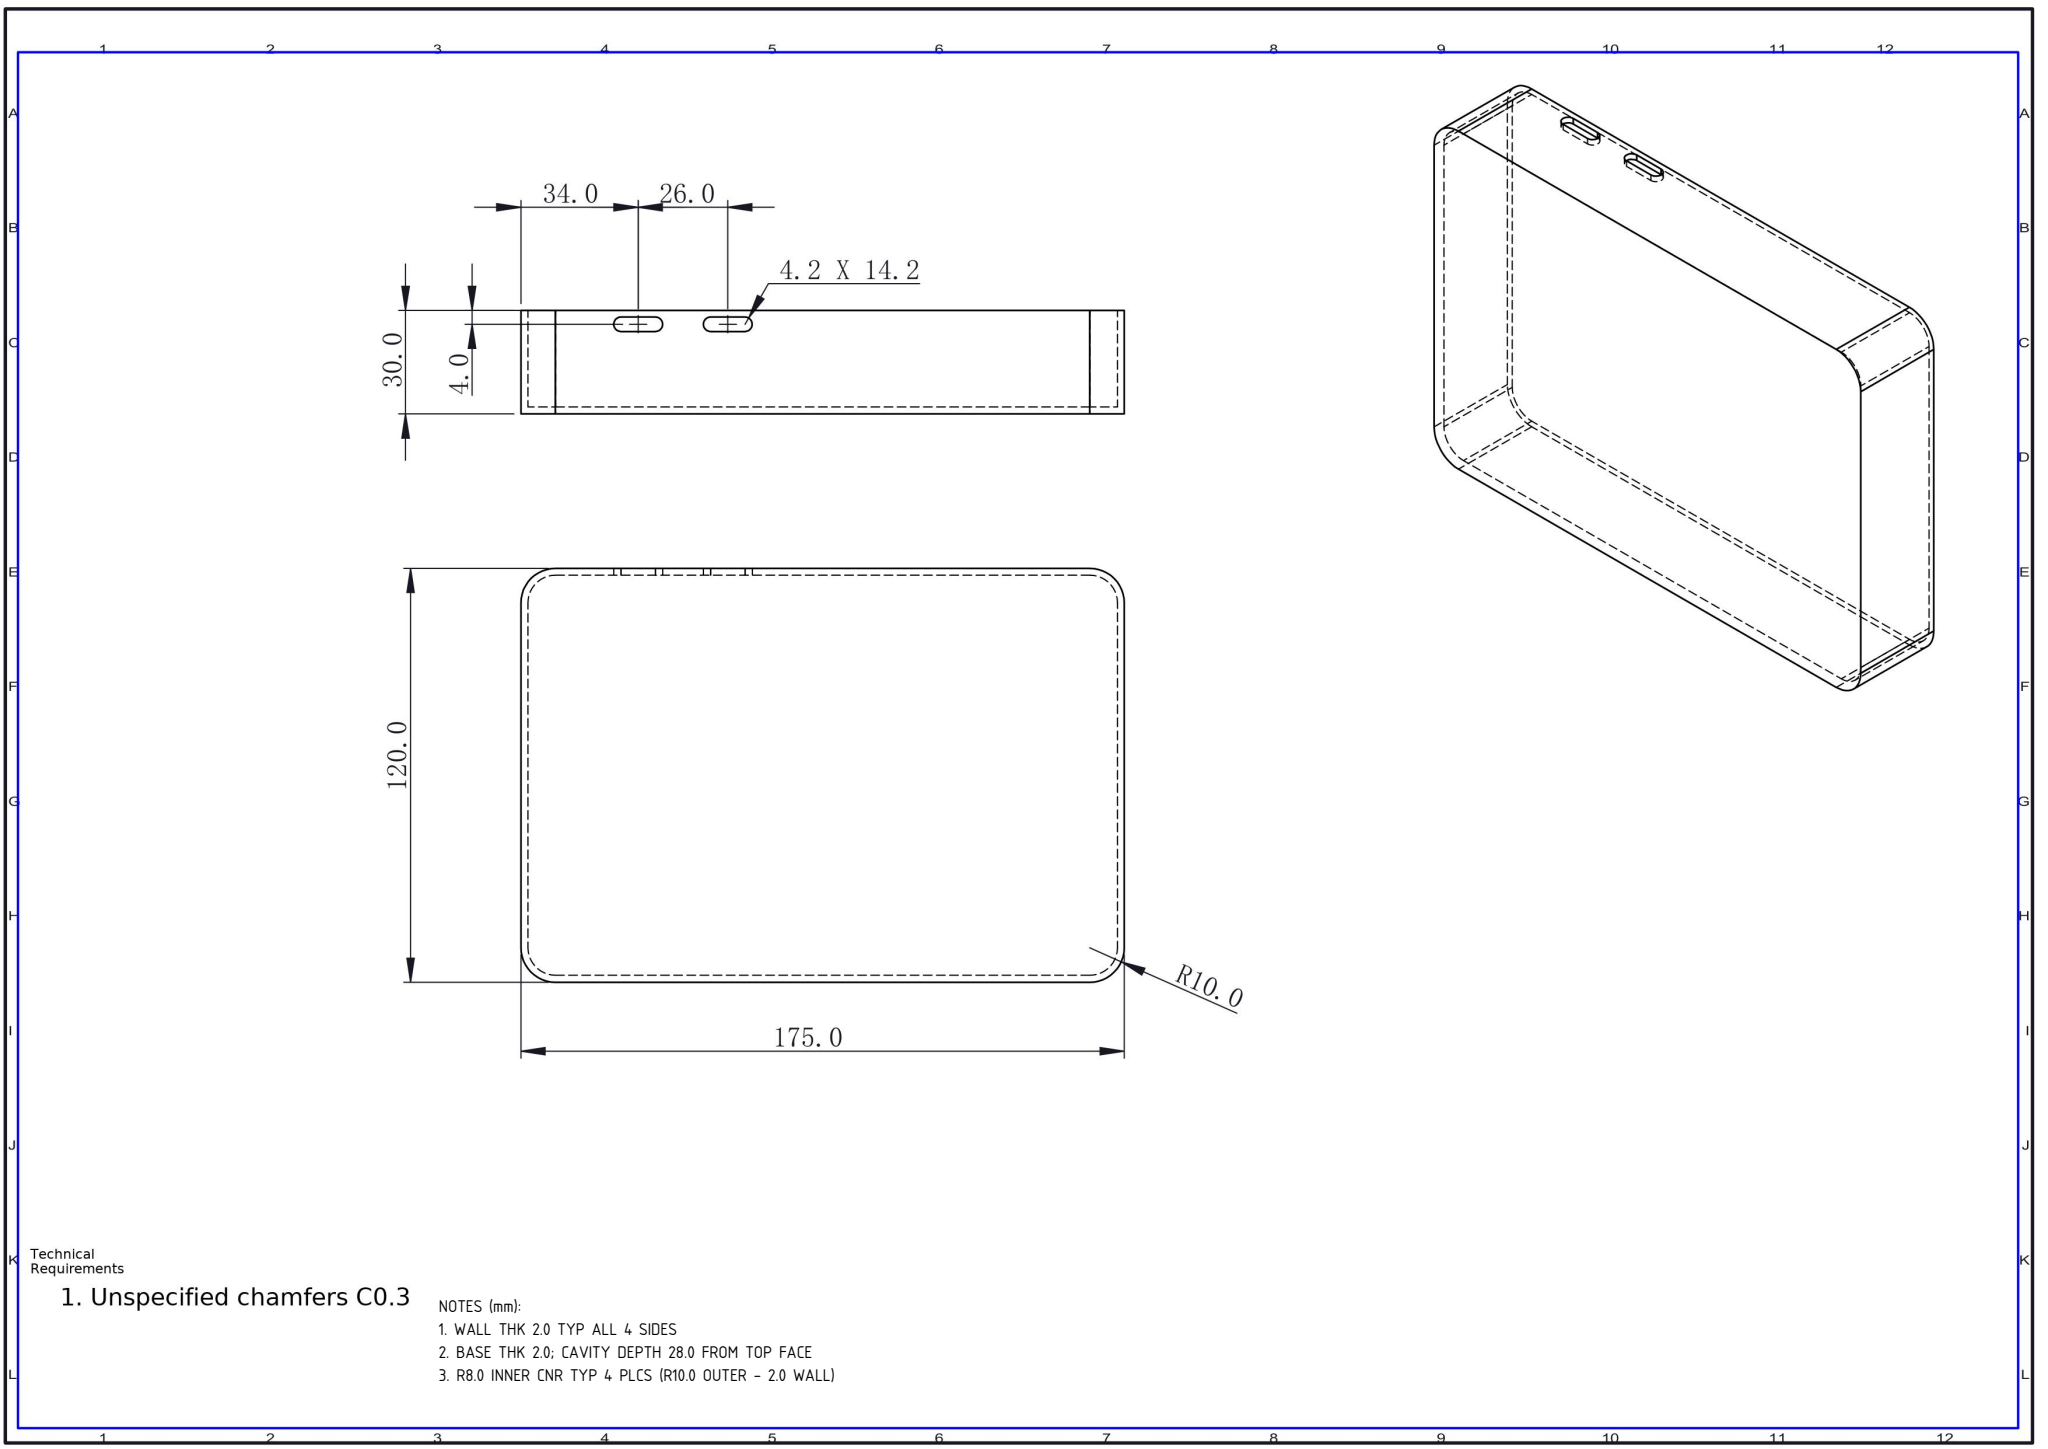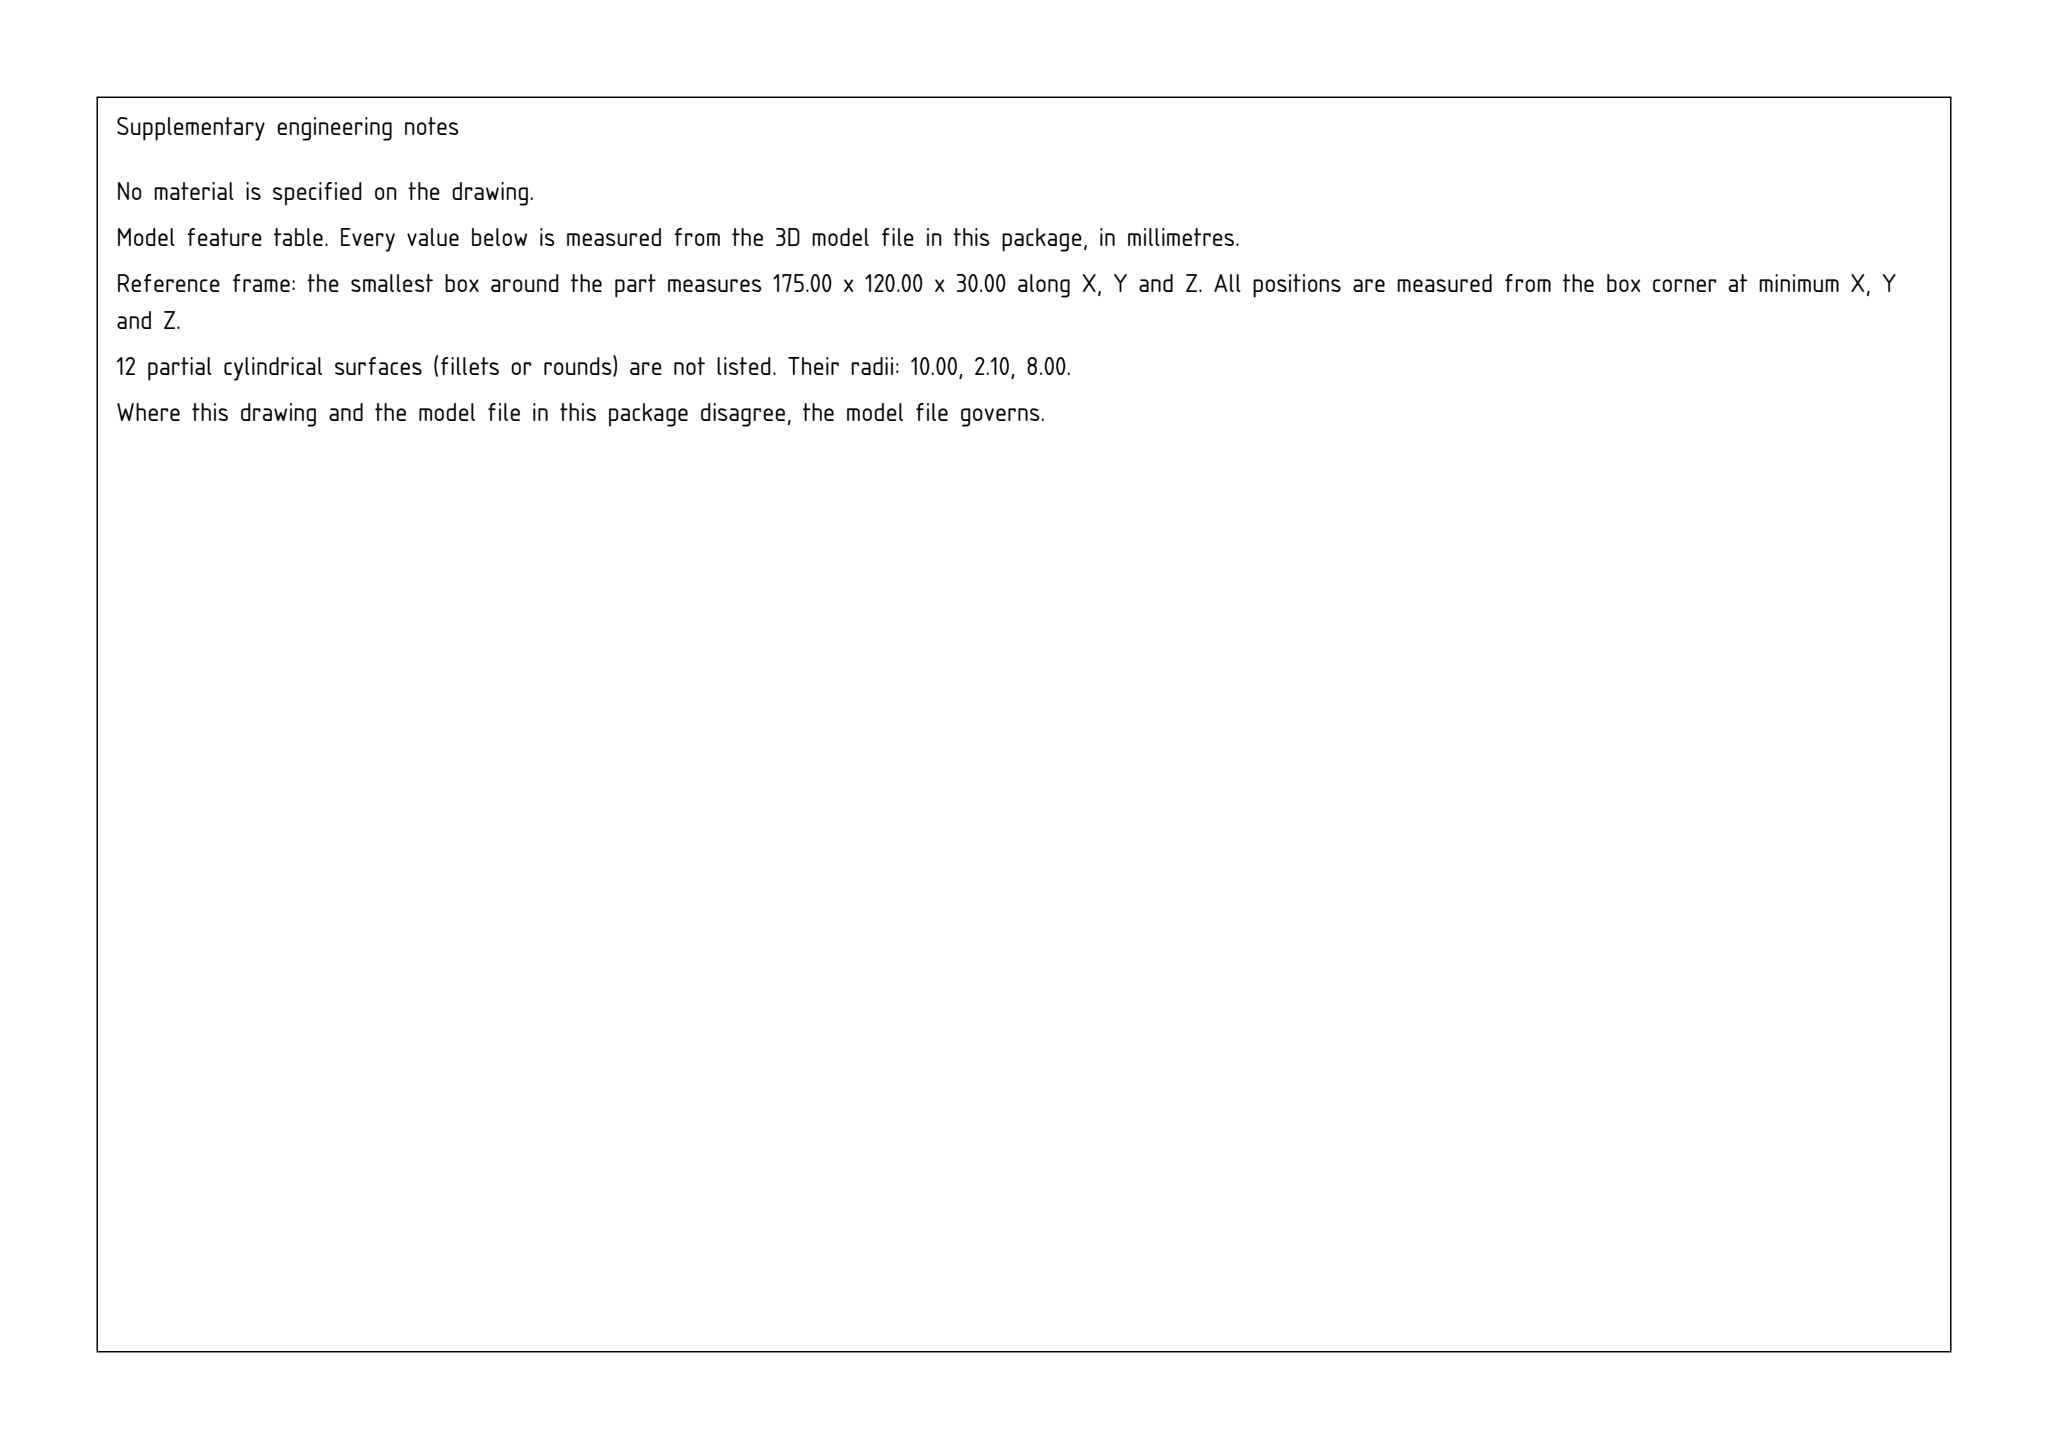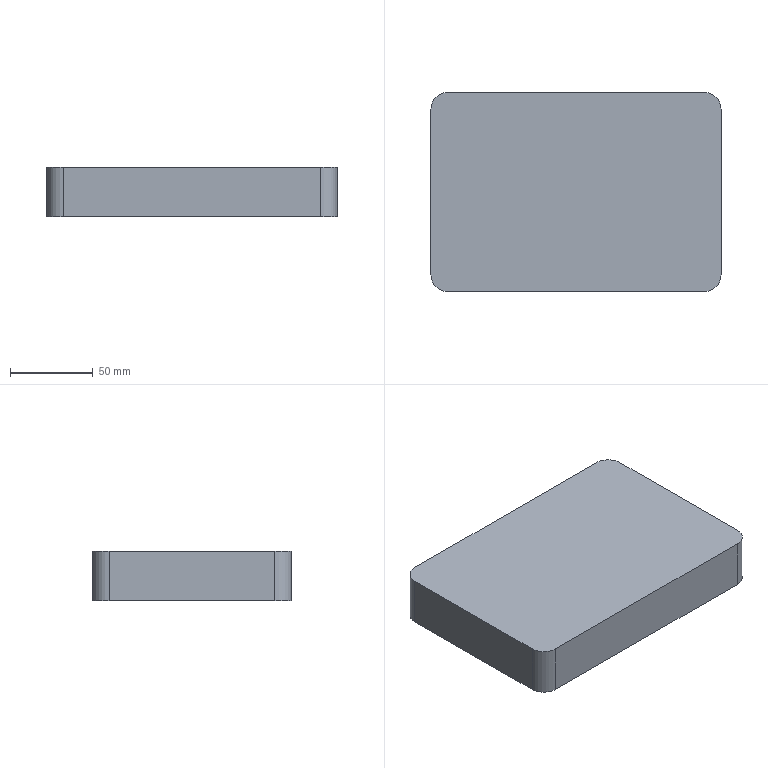Part | SolidWorks | mm | 1 solid | 27 faces | box 175 x 120 x 30 mm | volume 73332 mm3 | plane 15 | cylinder 12 | commonest cylinder face diameters 20 x4 16 x4 4.2 x4
Drawing notes:
WALL THK 2.0 TYP ALL 4 SIDES | from the solid: x-planes 0/2.0 & 173.0/175.0; y-planes 0/2.0 & 118.0/120.0 (bbox 175x120)
BASE THK 2.0; CAVITY DEPTH 28.0 FROM TOP FACE | from the solid: z-planes 0, 28.0 and 30.0; cavity cyls len 28.0 from z=2.0 to z=30.0
R8.0 INNER CNR TYP 4 PLCS (R10.0 OUTER - 2.0 WALL) | from the solid: dia 16.0 z-axis cyls at (10,10),(10,110),(165,10),(165,110) = R8.0; outer dia 20.0 = R10.0
build123d program:
from build123d import *

# Parameters (mm, degrees)
SKETCH1_W           = 175
SKETCH1_H           = 120
BOSS_EXTRUDE1_DEPTH = 30
FILLET1_R           = 10
SHELL1_T            = -2
CUT_EXTRUDE1_REACH  = 216.301


with BuildPart() as part:
    # Sketch1 → Boss-Extrude1 (new body)
    with BuildSketch(Plane.XY):
        with Locations((87.5, -60)):
            Rectangle(SKETCH1_W, SKETCH1_H)
    extrude(amount=BOSS_EXTRUDE1_DEPTH)

    # Fillet1
    fillet1_edges = [part.edges().sort_by_distance(p)[0] for p in [
        (0, 0, 15),
        (175, 0, 15),
        (175, -120, 15),
        (0, -120, 15),
    ]]
    fillet(fillet1_edges, radius=FILLET1_R)

    # Shell1
    shell1_openings = [part.faces().sort_by_distance(p)[0] for p in [
        (87.5, -60, 0),
    ]]
    offset(amount=SHELL1_T, openings=shell1_openings, kind=Kind.INTERSECTION)

    # Sketch2 → Cut-Extrude1 (cut, up to next)
    with BuildSketch(Plane(origin=(0, 0, 0), x_dir=(1, 0, 0), z_dir=(0, 1, 0)), mode=Mode.PRIVATE) as cut_extrude1_sk1:
        with BuildLine():
            Line((29, -1.9), (39, -1.9))
            ThreePointArc((39, -1.9), (41.1, -4), (39, -6.1))
            Line((39, -6.1), (29, -6.1))
            ThreePointArc((29, -6.1), (26.9, -4), (29, -1.9))
        make_face()
    cut_extrude1_tool1 = extrude(cut_extrude1_sk1.sketch, amount=-CUT_EXTRUDE1_REACH, mode=Mode.PRIVATE) & part.part
    # Sketch2 → Cut-Extrude1 (cut, up to next)
    with BuildSketch(Plane(origin=(0, 0, 0), x_dir=(1, 0, 0), z_dir=(0, 1, 0)), mode=Mode.PRIVATE) as cut_extrude1_sk2:
        with BuildLine():
            Line((55, -1.9), (65, -1.9))
            ThreePointArc((65, -1.9), (67.1, -4), (65, -6.1))
            Line((65, -6.1), (55, -6.1))
            ThreePointArc((55, -6.1), (52.9, -4), (55, -1.9))
        make_face()
    cut_extrude1_tool2 = extrude(cut_extrude1_sk2.sketch, amount=-CUT_EXTRUDE1_REACH, mode=Mode.PRIVATE) & part.part
    add(cut_extrude1_tool1.solids().sort_by_distance((34, 0, 4))[0], mode=Mode.SUBTRACT)
    add(cut_extrude1_tool2.solids().sort_by_distance((60, 0, 4))[0], mode=Mode.SUBTRACT)


solid = part.part
STEP:
#1=CARTESIAN_POINT('',(165.,0.,0.));
#2=VERTEX_POINT('',#1);
#3=CARTESIAN_POINT('',(10.,0.,0.));
#4=VERTEX_POINT('',#3);
#5=CARTESIAN_POINT('',(0.,0.,0.));
#6=DIRECTION('',(-1.,0.,0.));
#7=VECTOR('',#6,1000.);
#8=LINE('',#5,#7);
#9=EDGE_CURVE('',#2,#4,#8,.T.);
#10=ORIENTED_EDGE('',*,*,#9,.F.);
#11=CARTESIAN_POINT('',(175.,-10.,0.));
#12=VERTEX_POINT('',#11);
#13=CARTESIAN_POINT('',(165.,-10.,0.));
#14=DIRECTION('',(0.,0.,-1.));
#15=DIRECTION('',(1.,-0.,0.));
#16=AXIS2_PLACEMENT_3D('',#13,#14,#15);
#17=CIRCLE('',#16,10.);
#18=EDGE_CURVE('',#2,#12,#17,.T.);
#19=ORIENTED_EDGE('',*,*,#18,.T.);
#20=CARTESIAN_POINT('',(175.,-110.,0.));
#21=VERTEX_POINT('',#20);
#22=CARTESIAN_POINT('',(175.,0.,0.));
#23=DIRECTION('',(-0.,1.,0.));
#24=VECTOR('',#23,1000.);
#25=LINE('',#22,#24);
#26=EDGE_CURVE('',#21,#12,#25,.T.);
#27=ORIENTED_EDGE('',*,*,#26,.F.);
#28=CARTESIAN_POINT('',(165.,-120.,0.));
#29=VERTEX_POINT('',#28);
#30=CARTESIAN_POINT('',(165.,-110.,0.));
#31=DIRECTION('',(0.,0.,-1.));
#32=DIRECTION('',(1.,0.,0.));
#33=AXIS2_PLACEMENT_3D('',#30,#31,#32);
#34=CIRCLE('',#33,10.);
#35=EDGE_CURVE('',#21,#29,#34,.T.);
#36=ORIENTED_EDGE('',*,*,#35,.T.);
#37=CARTESIAN_POINT('',(10.,-120.,0.));
#38=VERTEX_POINT('',#37);
#39=CARTESIAN_POINT('',(0.,-120.,0.));
#40=DIRECTION('',(1.,0.,0.));
#41=VECTOR('',#40,1000.);
#42=LINE('',#39,#41);
#43=EDGE_CURVE('',#38,#29,#42,.T.);
#44=ORIENTED_EDGE('',*,*,#43,.F.);
#45=CARTESIAN_POINT('',(0.,-110.,0.));
#46=VERTEX_POINT('',#45);
#47=CARTESIAN_POINT('',(10.,-110.,0.));
#48=DIRECTION('',(0.,0.,-1.));
#49=DIRECTION('',(1.,0.,0.));
#50=AXIS2_PLACEMENT_3D('',#47,#48,#49);
#51=CIRCLE('',#50,10.);
#52=EDGE_CURVE('',#38,#46,#51,.T.);
#53=ORIENTED_EDGE('',*,*,#52,.T.);
#54=CARTESIAN_POINT('',(0.,-10.,0.));
#55=VERTEX_POINT('',#54);
#56=CARTESIAN_POINT('',(0.,0.,0.));
#57=DIRECTION('',(0.,-1.,0.));
#58=VECTOR('',#57,1000.);
#59=LINE('',#56,#58);
#60=EDGE_CURVE('',#55,#46,#59,.T.);
#61=ORIENTED_EDGE('',*,*,#60,.F.);
#62=CARTESIAN_POINT('',(10.,-10.,0.));
#63=DIRECTION('',(0.,0.,-1.));
#64=DIRECTION('',(1.,0.,0.));
#65=AXIS2_PLACEMENT_3D('',#62,#63,#64);
#66=CIRCLE('',#65,10.);
#67=EDGE_CURVE('',#55,#4,#66,.T.);
#68=ORIENTED_EDGE('',*,*,#67,.T.);
#69=EDGE_LOOP('',(#10,#19,#27,#36,#44,#53,#61,#68));
#70=FACE_OUTER_BOUND('',#69,.T.);
#71=CARTESIAN_POINT('',(165.,-2.,0.));
#72=VERTEX_POINT('',#71);
#73=CARTESIAN_POINT('',(173.,-10.,0.));
#74=VERTEX_POINT('',#73);
#75=CARTESIAN_POINT('',(165.,-10.,0.));
#76=DIRECTION('',(0.,0.,-1.));
#77=DIRECTION('',(1.,-0.,0.));
#78=AXIS2_PLACEMENT_3D('',#75,#76,#77);
#79=CIRCLE('',#78,8.);
#80=EDGE_CURVE('',#72,#74,#79,.T.);
#81=ORIENTED_EDGE('',*,*,#80,.F.);
#82=CARTESIAN_POINT('',(10.,-2.,0.));
#83=VERTEX_POINT('',#82);
#84=CARTESIAN_POINT('',(0.,-2.,0.));
#85=DIRECTION('',(-1.,0.,0.));
#86=VECTOR('',#85,1000.);
#87=LINE('',#84,#86);
#88=EDGE_CURVE('',#72,#83,#87,.T.);
#89=ORIENTED_EDGE('',*,*,#88,.T.);
#90=CARTESIAN_POINT('',(2.,-10.,0.));
#91=VERTEX_POINT('',#90);
#92=CARTESIAN_POINT('',(10.,-10.,0.));
#93=DIRECTION('',(0.,0.,-1.));
#94=DIRECTION('',(1.,0.,0.));
#95=AXIS2_PLACEMENT_3D('',#92,#93,#94);
#96=CIRCLE('',#95,8.);
#97=EDGE_CURVE('',#91,#83,#96,.T.);
#98=ORIENTED_EDGE('',*,*,#97,.F.);
#99=CARTESIAN_POINT('',(2.,-110.,0.));
#100=VERTEX_POINT('',#99);
#101=CARTESIAN_POINT('',(2.,0.,0.));
#102=DIRECTION('',(0.,-1.,0.));
#103=VECTOR('',#102,1000.);
#104=LINE('',#101,#103);
#105=EDGE_CURVE('',#91,#100,#104,.T.);
#106=ORIENTED_EDGE('',*,*,#105,.T.);
#107=CARTESIAN_POINT('',(10.,-118.,0.));
#108=VERTEX_POINT('',#107);
#109=CARTESIAN_POINT('',(10.,-110.,0.));
#110=DIRECTION('',(0.,0.,-1.));
#111=DIRECTION('',(1.,0.,0.));
#112=AXIS2_PLACEMENT_3D('',#109,#110,#111);
#113=CIRCLE('',#112,8.);
#114=EDGE_CURVE('',#108,#100,#113,.T.);
#115=ORIENTED_EDGE('',*,*,#114,.F.);
#116=CARTESIAN_POINT('',(165.,-118.,0.));
#117=VERTEX_POINT('',#116);
#118=CARTESIAN_POINT('',(0.,-118.,0.));
#119=DIRECTION('',(1.,0.,0.));
#120=VECTOR('',#119,1000.);
#121=LINE('',#118,#120);
#122=EDGE_CURVE('',#108,#117,#121,.T.);
#123=ORIENTED_EDGE('',*,*,#122,.T.);
#124=CARTESIAN_POINT('',(173.,-110.,0.));
#125=VERTEX_POINT('',#124);
#126=CARTESIAN_POINT('',(165.,-110.,0.));
#127=DIRECTION('',(0.,0.,-1.));
#128=DIRECTION('',(1.,0.,0.));
#129=AXIS2_PLACEMENT_3D('',#126,#127,#128);
#130=CIRCLE('',#129,8.);
#131=EDGE_CURVE('',#125,#117,#130,.T.);
#132=ORIENTED_EDGE('',*,*,#131,.F.);
#133=CARTESIAN_POINT('',(173.,-0.,0.));
#134=DIRECTION('',(-0.,1.,0.));
#135=VECTOR('',#134,1000.);
#136=LINE('',#133,#135);
#137=EDGE_CURVE('',#125,#74,#136,.T.);
#138=ORIENTED_EDGE('',*,*,#137,.T.);
#139=EDGE_LOOP('',(#81,#89,#98,#106,#115,#123,#132,#138));
#140=FACE_BOUND('',#139,.T.);
#141=CARTESIAN_POINT('',(0.,0.,0.));
#142=DIRECTION('',(0.,0.,1.));
#143=DIRECTION('',(1.,0.,0.));
#144=AXIS2_PLACEMENT_3D('',#141,#142,#143);
#145=PLANE('',#144);
#146=ADVANCED_FACE('',(#70,#140),#145,.F.);
#147=CARTESIAN_POINT('',(0.,-10.,30.));
#148=VERTEX_POINT('',#147);
#149=CARTESIAN_POINT('',(0.,-110.,30.));
#150=VERTEX_POINT('',#149);
#151=CARTESIAN_POINT('',(0.,0.,30.));
#152=DIRECTION('',(0.,-1.,0.));
#153=VECTOR('',#152,1000.);
#154=LINE('',#151,#153);
#155=EDGE_CURVE('',#148,#150,#154,.T.);
#156=ORIENTED_EDGE('',*,*,#155,.F.);
#157=CARTESIAN_POINT('',(0.,-10.,30.));
#158=DIRECTION('',(0.,0.,-1.));
#159=VECTOR('',#158,1000.);
#160=LINE('',#157,#159);
#161=EDGE_CURVE('',#148,#55,#160,.T.);
#162=ORIENTED_EDGE('',*,*,#161,.T.);
#163=ORIENTED_EDGE('',*,*,#60,.T.);
#164=CARTESIAN_POINT('',(0.,-110.,30.));
#165=DIRECTION('',(0.,0.,1.));
#166=VECTOR('',#165,1000.);
#167=LINE('',#164,#166);
#168=EDGE_CURVE('',#46,#150,#167,.T.);
#169=ORIENTED_EDGE('',*,*,#168,.T.);
#170=EDGE_LOOP('',(#156,#162,#163,#169));
#171=FACE_OUTER_BOUND('',#170,.T.);
#172=CARTESIAN_POINT('',(0.,0.,30.));
#173=DIRECTION('',(1.,0.,0.));
#174=DIRECTION('',(-0.,1.,0.));
#175=AXIS2_PLACEMENT_3D('',#172,#173,#174);
#176=PLANE('',#175);
#177=ADVANCED_FACE('',(#171),#176,.F.);
#178=ORIENTED_EDGE('',*,*,#43,.T.);
#179=CARTESIAN_POINT('',(165.,-120.,30.));
#180=VERTEX_POINT('',#179);
#181=CARTESIAN_POINT('',(165.,-120.,30.));
#182=DIRECTION('',(0.,0.,1.));
#183=VECTOR('',#182,1000.);
#184=LINE('',#181,#183);
#185=EDGE_CURVE('',#29,#180,#184,.T.);
#186=ORIENTED_EDGE('',*,*,#185,.T.);
#187=CARTESIAN_POINT('',(10.,-120.,30.));
#188=VERTEX_POINT('',#187);
#189=CARTESIAN_POINT('',(0.,-120.,30.));
#190=DIRECTION('',(1.,0.,0.));
#191=VECTOR('',#190,1000.);
#192=LINE('',#189,#191);
#193=EDGE_CURVE('',#188,#180,#192,.T.);
#194=ORIENTED_EDGE('',*,*,#193,.F.);
#195=CARTESIAN_POINT('',(10.,-120.,30.));
#196=DIRECTION('',(0.,0.,-1.));
#197=VECTOR('',#196,1000.);
#198=LINE('',#195,#197);
#199=EDGE_CURVE('',#188,#38,#198,.T.);
#200=ORIENTED_EDGE('',*,*,#199,.T.);
#201=EDGE_LOOP('',(#178,#186,#194,#200));
#202=FACE_OUTER_BOUND('',#201,.T.);
#203=CARTESIAN_POINT('',(0.,-120.,30.));
#204=DIRECTION('',(0.,1.,0.));
#205=DIRECTION('',(0.,0.,1.));
#206=AXIS2_PLACEMENT_3D('',#203,#204,#205);
#207=PLANE('',#206);
#208=ADVANCED_FACE('',(#202),#207,.F.);
#209=ORIENTED_EDGE('',*,*,#26,.T.);
#210=CARTESIAN_POINT('',(175.,-10.,30.));
#211=VERTEX_POINT('',#210);
#212=CARTESIAN_POINT('',(175.,-10.,30.));
#213=DIRECTION('',(0.,0.,1.));
#214=VECTOR('',#213,1000.);
#215=LINE('',#212,#214);
#216=EDGE_CURVE('',#12,#211,#215,.T.);
#217=ORIENTED_EDGE('',*,*,#216,.T.);
#218=CARTESIAN_POINT('',(175.,-110.,30.));
#219=VERTEX_POINT('',#218);
#220=CARTESIAN_POINT('',(175.,0.,30.));
#221=DIRECTION('',(-0.,1.,0.));
#222=VECTOR('',#221,1000.);
#223=LINE('',#220,#222);
#224=EDGE_CURVE('',#219,#211,#223,.T.);
#225=ORIENTED_EDGE('',*,*,#224,.F.);
#226=CARTESIAN_POINT('',(175.,-110.,30.));
#227=DIRECTION('',(0.,0.,-1.));
#228=VECTOR('',#227,1000.);
#229=LINE('',#226,#228);
#230=EDGE_CURVE('',#219,#21,#229,.T.);
#231=ORIENTED_EDGE('',*,*,#230,.T.);
#232=EDGE_LOOP('',(#209,#217,#225,#231));
#233=FACE_OUTER_BOUND('',#232,.T.);
#234=CARTESIAN_POINT('',(175.,0.,30.));
#235=DIRECTION('',(-1.,-0.,0.));
#236=DIRECTION('',(0.,-1.,0.));
#237=AXIS2_PLACEMENT_3D('',#234,#235,#236);
#238=PLANE('',#237);
#239=ADVANCED_FACE('',(#233),#238,.F.);
#240=CARTESIAN_POINT('',(39.,0.,6.1));
#241=VERTEX_POINT('',#240);
#242=CARTESIAN_POINT('',(39.,0.,1.9));
#243=VERTEX_POINT('',#242);
#244=CARTESIAN_POINT('',(39.,0.,4.));
#245=DIRECTION('',(0.,1.,0.));
#246=DIRECTION('',(0.,0.,1.));
#247=AXIS2_PLACEMENT_3D('',#244,#245,#246);
#248=CIRCLE('',#247,2.1);
#249=EDGE_CURVE('',#241,#243,#248,.T.);
#250=ORIENTED_EDGE('',*,*,#249,.F.);
#251=CARTESIAN_POINT('',(29.,0.,6.1));
#252=VERTEX_POINT('',#251);
#253=CARTESIAN_POINT('',(29.,0.,6.1));
#254=DIRECTION('',(1.,0.,-0.));
#255=VECTOR('',#254,1000.);
#256=LINE('',#253,#255);
#257=EDGE_CURVE('',#252,#241,#256,.T.);
#258=ORIENTED_EDGE('',*,*,#257,.F.);
#259=CARTESIAN_POINT('',(29.,0.,1.9));
#260=VERTEX_POINT('',#259);
#261=CARTESIAN_POINT('',(29.,0.,4.));
#262=DIRECTION('',(0.,1.,0.));
#263=DIRECTION('',(0.,0.,1.));
#264=AXIS2_PLACEMENT_3D('',#261,#262,#263);
#265=CIRCLE('',#264,2.1);
#266=EDGE_CURVE('',#260,#252,#265,.T.);
#267=ORIENTED_EDGE('',*,*,#266,.F.);
#268=CARTESIAN_POINT('',(29.,0.,1.9));
#269=DIRECTION('',(-1.,0.,0.));
#270=VECTOR('',#269,1000.);
#271=LINE('',#268,#270);
#272=EDGE_CURVE('',#243,#260,#271,.T.);
#273=ORIENTED_EDGE('',*,*,#272,.F.);
#274=EDGE_LOOP('',(#250,#258,#267,#273));
#275=FACE_BOUND('',#274,.T.);
#276=CARTESIAN_POINT('',(65.,0.,6.1));
#277=VERTEX_POINT('',#276);
#278=CARTESIAN_POINT('',(65.,0.,1.9));
#279=VERTEX_POINT('',#278);
#280=CARTESIAN_POINT('',(65.,0.,4.));
#281=DIRECTION('',(0.,1.,0.));
#282=DIRECTION('',(0.,0.,1.));
#283=AXIS2_PLACEMENT_3D('',#280,#281,#282);
#284=CIRCLE('',#283,2.1);
#285=EDGE_CURVE('',#277,#279,#284,.T.);
#286=ORIENTED_EDGE('',*,*,#285,.F.);
#287=CARTESIAN_POINT('',(55.,0.,6.1));
#288=VERTEX_POINT('',#287);
#289=CARTESIAN_POINT('',(55.,0.,6.1));
#290=DIRECTION('',(1.,0.,-0.));
#291=VECTOR('',#290,1000.);
#292=LINE('',#289,#291);
#293=EDGE_CURVE('',#288,#277,#292,.T.);
#294=ORIENTED_EDGE('',*,*,#293,.F.);
#295=CARTESIAN_POINT('',(55.,0.,1.9));
#296=VERTEX_POINT('',#295);
#297=CARTESIAN_POINT('',(55.,0.,4.));
#298=DIRECTION('',(0.,1.,0.));
#299=DIRECTION('',(0.,0.,1.));
#300=AXIS2_PLACEMENT_3D('',#297,#298,#299);
#301=CIRCLE('',#300,2.1);
#302=EDGE_CURVE('',#296,#288,#301,.T.);
#303=ORIENTED_EDGE('',*,*,#302,.F.);
#304=CARTESIAN_POINT('',(55.,0.,1.9));
#305=DIRECTION('',(-1.,0.,0.));
#306=VECTOR('',#305,1000.);
#307=LINE('',#304,#306);
#308=EDGE_CURVE('',#279,#296,#307,.T.);
#309=ORIENTED_EDGE('',*,*,#308,.F.);
#310=EDGE_LOOP('',(#286,#294,#303,#309));
#311=FACE_BOUND('',#310,.T.);
#312=CARTESIAN_POINT('',(165.,0.,30.));
#313=VERTEX_POINT('',#312);
#314=CARTESIAN_POINT('',(10.,0.,30.));
#315=VERTEX_POINT('',#314);
#316=CARTESIAN_POINT('',(0.,0.,30.));
#317=DIRECTION('',(-1.,0.,0.));
#318=VECTOR('',#317,1000.);
#319=LINE('',#316,#318);
#320=EDGE_CURVE('',#313,#315,#319,.T.);
#321=ORIENTED_EDGE('',*,*,#320,.F.);
#322=CARTESIAN_POINT('',(165.,0.,30.));
#323=DIRECTION('',(0.,0.,-1.));
#324=VECTOR('',#323,1000.);
#325=LINE('',#322,#324);
#326=EDGE_CURVE('',#313,#2,#325,.T.);
#327=ORIENTED_EDGE('',*,*,#326,.T.);
#328=ORIENTED_EDGE('',*,*,#9,.T.);
#329=CARTESIAN_POINT('',(10.,0.,30.));
#330=DIRECTION('',(0.,0.,1.));
#331=VECTOR('',#330,1000.);
#332=LINE('',#329,#331);
#333=EDGE_CURVE('',#4,#315,#332,.T.);
#334=ORIENTED_EDGE('',*,*,#333,.T.);
#335=EDGE_LOOP('',(#321,#327,#328,#334));
#336=FACE_OUTER_BOUND('',#335,.T.);
#337=CARTESIAN_POINT('',(0.,0.,30.));
#338=DIRECTION('',(0.,-1.,0.));
#339=DIRECTION('',(0.,0.,-1.));
#340=AXIS2_PLACEMENT_3D('',#337,#338,#339);
#341=PLANE('',#340);
#342=ADVANCED_FACE('',(#275,#311,#336),#341,.F.);
#343=ORIENTED_EDGE('',*,*,#224,.T.);
#344=CARTESIAN_POINT('',(165.,-10.,30.));
#345=DIRECTION('',(0.,0.,1.));
#346=DIRECTION('',(1.,0.,0.));
#347=AXIS2_PLACEMENT_3D('',#344,#345,#346);
#348=CIRCLE('',#347,10.);
#349=EDGE_CURVE('',#211,#313,#348,.T.);
#350=ORIENTED_EDGE('',*,*,#349,.T.);
#351=ORIENTED_EDGE('',*,*,#320,.T.);
#352=CARTESIAN_POINT('',(10.,-10.,30.));
#353=DIRECTION('',(0.,0.,1.));
#354=DIRECTION('',(1.,0.,0.));
#355=AXIS2_PLACEMENT_3D('',#352,#353,#354);
#356=CIRCLE('',#355,10.);
#357=EDGE_CURVE('',#315,#148,#356,.T.);
#358=ORIENTED_EDGE('',*,*,#357,.T.);
#359=ORIENTED_EDGE('',*,*,#155,.T.);
#360=CARTESIAN_POINT('',(10.,-110.,30.));
#361=DIRECTION('',(0.,0.,1.));
#362=DIRECTION('',(1.,0.,0.));
#363=AXIS2_PLACEMENT_3D('',#360,#361,#362);
#364=CIRCLE('',#363,10.);
#365=EDGE_CURVE('',#150,#188,#364,.T.);
#366=ORIENTED_EDGE('',*,*,#365,.T.);
#367=ORIENTED_EDGE('',*,*,#193,.T.);
#368=CARTESIAN_POINT('',(165.,-110.,30.));
#369=DIRECTION('',(0.,0.,1.));
#370=DIRECTION('',(1.,0.,0.));
#371=AXIS2_PLACEMENT_3D('',#368,#369,#370);
#372=CIRCLE('',#371,10.);
#373=EDGE_CURVE('',#180,#219,#372,.T.);
#374=ORIENTED_EDGE('',*,*,#373,.T.);
#375=EDGE_LOOP('',(#343,#350,#351,#358,#359,#366,#367,#374));
#376=FACE_OUTER_BOUND('',#375,.T.);
#377=CARTESIAN_POINT('',(0.,0.,30.));
#378=DIRECTION('',(0.,0.,1.));
#379=DIRECTION('',(1.,0.,0.));
#380=AXIS2_PLACEMENT_3D('',#377,#378,#379);
#381=PLANE('',#380);
#382=ADVANCED_FACE('',(#376),#381,.T.);
#383=ORIENTED_EDGE('',*,*,#349,.F.);
#384=ORIENTED_EDGE('',*,*,#216,.F.);
#385=ORIENTED_EDGE('',*,*,#18,.F.);
#386=ORIENTED_EDGE('',*,*,#326,.F.);
#387=EDGE_LOOP('',(#383,#384,#385,#386));
#388=FACE_OUTER_BOUND('',#387,.T.);
#389=CARTESIAN_POINT('',(165.,-10.,30.));
#390=DIRECTION('',(0.,0.,-1.));
#391=DIRECTION('',(-1.,0.,0.));
#392=AXIS2_PLACEMENT_3D('',#389,#390,#391);
#393=CYLINDRICAL_SURFACE('',#392,10.);
#394=ADVANCED_FACE('',(#388),#393,.T.);
#395=ORIENTED_EDGE('',*,*,#357,.F.);
#396=ORIENTED_EDGE('',*,*,#333,.F.);
#397=ORIENTED_EDGE('',*,*,#67,.F.);
#398=ORIENTED_EDGE('',*,*,#161,.F.);
#399=EDGE_LOOP('',(#395,#396,#397,#398));
#400=FACE_OUTER_BOUND('',#399,.T.);
#401=CARTESIAN_POINT('',(10.,-10.,30.));
#402=DIRECTION('',(0.,0.,-1.));
#403=DIRECTION('',(-1.,0.,0.));
#404=AXIS2_PLACEMENT_3D('',#401,#402,#403);
#405=CYLINDRICAL_SURFACE('',#404,10.);
#406=ADVANCED_FACE('',(#400),#405,.T.);
#407=ORIENTED_EDGE('',*,*,#373,.F.);
#408=ORIENTED_EDGE('',*,*,#185,.F.);
#409=ORIENTED_EDGE('',*,*,#35,.F.);
#410=ORIENTED_EDGE('',*,*,#230,.F.);
#411=EDGE_LOOP('',(#407,#408,#409,#410));
#412=FACE_OUTER_BOUND('',#411,.T.);
#413=CARTESIAN_POINT('',(165.,-110.,30.));
#414=DIRECTION('',(0.,0.,-1.));
#415=DIRECTION('',(-1.,0.,0.));
#416=AXIS2_PLACEMENT_3D('',#413,#414,#415);
#417=CYLINDRICAL_SURFACE('',#416,10.);
#418=ADVANCED_FACE('',(#412),#417,.T.);
#419=ORIENTED_EDGE('',*,*,#365,.F.);
#420=ORIENTED_EDGE('',*,*,#168,.F.);
#421=ORIENTED_EDGE('',*,*,#52,.F.);
#422=ORIENTED_EDGE('',*,*,#199,.F.);
#423=EDGE_LOOP('',(#419,#420,#421,#422));
#424=FACE_OUTER_BOUND('',#423,.T.);
#425=CARTESIAN_POINT('',(10.,-110.,30.));
#426=DIRECTION('',(0.,0.,-1.));
#427=DIRECTION('',(-1.,0.,0.));
#428=AXIS2_PLACEMENT_3D('',#425,#426,#427);
#429=CYLINDRICAL_SURFACE('',#428,10.);
#430=ADVANCED_FACE('',(#424),#429,.T.);
#431=CARTESIAN_POINT('',(2.,-10.,28.));
#432=VERTEX_POINT('',#431);
#433=CARTESIAN_POINT('',(2.,-110.,28.));
#434=VERTEX_POINT('',#433);
#435=CARTESIAN_POINT('',(2.,0.,28.));
#436=DIRECTION('',(0.,-1.,0.));
#437=VECTOR('',#436,1000.);
#438=LINE('',#435,#437);
#439=EDGE_CURVE('',#432,#434,#438,.T.);
#440=ORIENTED_EDGE('',*,*,#439,.T.);
#441=CARTESIAN_POINT('',(2.,-110.,30.));
#442=DIRECTION('',(0.,0.,1.));
#443=VECTOR('',#442,1000.);
#444=LINE('',#441,#443);
#445=EDGE_CURVE('',#100,#434,#444,.T.);
#446=ORIENTED_EDGE('',*,*,#445,.F.);
#447=ORIENTED_EDGE('',*,*,#105,.F.);
#448=CARTESIAN_POINT('',(2.,-10.,30.));
#449=DIRECTION('',(0.,0.,-1.));
#450=VECTOR('',#449,1000.);
#451=LINE('',#448,#450);
#452=EDGE_CURVE('',#432,#91,#451,.T.);
#453=ORIENTED_EDGE('',*,*,#452,.F.);
#454=EDGE_LOOP('',(#440,#446,#447,#453));
#455=FACE_OUTER_BOUND('',#454,.T.);
#456=CARTESIAN_POINT('',(2.,0.,30.));
#457=DIRECTION('',(1.,0.,0.));
#458=DIRECTION('',(-0.,1.,0.));
#459=AXIS2_PLACEMENT_3D('',#456,#457,#458);
#460=PLANE('',#459);
#461=ADVANCED_FACE('',(#455),#460,.T.);
#462=ORIENTED_EDGE('',*,*,#122,.F.);
#463=CARTESIAN_POINT('',(10.,-118.,28.));
#464=VERTEX_POINT('',#463);
#465=CARTESIAN_POINT('',(10.,-118.,30.));
#466=DIRECTION('',(0.,0.,-1.));
#467=VECTOR('',#466,1000.);
#468=LINE('',#465,#467);
#469=EDGE_CURVE('',#464,#108,#468,.T.);
#470=ORIENTED_EDGE('',*,*,#469,.F.);
#471=CARTESIAN_POINT('',(165.,-118.,28.));
#472=VERTEX_POINT('',#471);
#473=CARTESIAN_POINT('',(0.,-118.,28.));
#474=DIRECTION('',(1.,0.,0.));
#475=VECTOR('',#474,1000.);
#476=LINE('',#473,#475);
#477=EDGE_CURVE('',#464,#472,#476,.T.);
#478=ORIENTED_EDGE('',*,*,#477,.T.);
#479=CARTESIAN_POINT('',(165.,-118.,30.));
#480=DIRECTION('',(0.,0.,1.));
#481=VECTOR('',#480,1000.);
#482=LINE('',#479,#481);
#483=EDGE_CURVE('',#117,#472,#482,.T.);
#484=ORIENTED_EDGE('',*,*,#483,.F.);
#485=EDGE_LOOP('',(#462,#470,#478,#484));
#486=FACE_OUTER_BOUND('',#485,.T.);
#487=CARTESIAN_POINT('',(0.,-118.,30.));
#488=DIRECTION('',(0.,1.,0.));
#489=DIRECTION('',(0.,0.,1.));
#490=AXIS2_PLACEMENT_3D('',#487,#488,#489);
#491=PLANE('',#490);
#492=ADVANCED_FACE('',(#486),#491,.T.);
#493=ORIENTED_EDGE('',*,*,#137,.F.);
#494=CARTESIAN_POINT('',(173.,-110.,28.));
#495=VERTEX_POINT('',#494);
#496=CARTESIAN_POINT('',(173.,-110.,30.));
#497=DIRECTION('',(0.,0.,-1.));
#498=VECTOR('',#497,1000.);
#499=LINE('',#496,#498);
#500=EDGE_CURVE('',#495,#125,#499,.T.);
#501=ORIENTED_EDGE('',*,*,#500,.F.);
#502=CARTESIAN_POINT('',(173.,-10.,28.));
#503=VERTEX_POINT('',#502);
#504=CARTESIAN_POINT('',(173.,-0.,28.));
#505=DIRECTION('',(-0.,1.,0.));
#506=VECTOR('',#505,1000.);
#507=LINE('',#504,#506);
#508=EDGE_CURVE('',#495,#503,#507,.T.);
#509=ORIENTED_EDGE('',*,*,#508,.T.);
#510=CARTESIAN_POINT('',(173.,-10.,30.));
#511=DIRECTION('',(0.,0.,1.));
#512=VECTOR('',#511,1000.);
#513=LINE('',#510,#512);
#514=EDGE_CURVE('',#74,#503,#513,.T.);
#515=ORIENTED_EDGE('',*,*,#514,.F.);
#516=EDGE_LOOP('',(#493,#501,#509,#515));
#517=FACE_OUTER_BOUND('',#516,.T.);
#518=CARTESIAN_POINT('',(173.,-0.,30.));
#519=DIRECTION('',(-1.,-0.,0.));
#520=DIRECTION('',(0.,-1.,0.));
#521=AXIS2_PLACEMENT_3D('',#518,#519,#520);
#522=PLANE('',#521);
#523=ADVANCED_FACE('',(#517),#522,.T.);
#524=CARTESIAN_POINT('',(29.,-2.,6.1));
#525=VERTEX_POINT('',#524);
#526=CARTESIAN_POINT('',(39.,-2.,6.1));
#527=VERTEX_POINT('',#526);
#528=CARTESIAN_POINT('',(29.,-2.,6.1));
#529=DIRECTION('',(1.,0.,-0.));
#530=VECTOR('',#529,1000.);
#531=LINE('',#528,#530);
#532=EDGE_CURVE('',#525,#527,#531,.T.);
#533=ORIENTED_EDGE('',*,*,#532,.T.);
#534=CARTESIAN_POINT('',(39.,-2.,1.9));
#535=VERTEX_POINT('',#534);
#536=CARTESIAN_POINT('',(39.,-2.,4.));
#537=DIRECTION('',(0.,1.,0.));
#538=DIRECTION('',(0.,0.,-1.));
#539=AXIS2_PLACEMENT_3D('',#536,#537,#538);
#540=CIRCLE('',#539,2.1);
#541=EDGE_CURVE('',#527,#535,#540,.T.);
#542=ORIENTED_EDGE('',*,*,#541,.T.);
#543=CARTESIAN_POINT('',(29.,-2.,1.9));
#544=VERTEX_POINT('',#543);
#545=CARTESIAN_POINT('',(29.,-2.,1.9));
#546=DIRECTION('',(-1.,0.,0.));
#547=VECTOR('',#546,1000.);
#548=LINE('',#545,#547);
#549=EDGE_CURVE('',#535,#544,#548,.T.);
#550=ORIENTED_EDGE('',*,*,#549,.T.);
#551=CARTESIAN_POINT('',(29.,-2.,4.));
#552=DIRECTION('',(0.,1.,0.));
#553=DIRECTION('',(0.,0.,-1.));
#554=AXIS2_PLACEMENT_3D('',#551,#552,#553);
#555=CIRCLE('',#554,2.1);
#556=EDGE_CURVE('',#544,#525,#555,.T.);
#557=ORIENTED_EDGE('',*,*,#556,.T.);
#558=EDGE_LOOP('',(#533,#542,#550,#557));
#559=FACE_BOUND('',#558,.T.);
#560=CARTESIAN_POINT('',(55.,-2.,6.1));
#561=VERTEX_POINT('',#560);
#562=CARTESIAN_POINT('',(65.,-2.,6.1));
#563=VERTEX_POINT('',#562);
#564=CARTESIAN_POINT('',(55.,-2.,6.1));
#565=DIRECTION('',(1.,0.,-0.));
#566=VECTOR('',#565,1000.);
#567=LINE('',#564,#566);
#568=EDGE_CURVE('',#561,#563,#567,.T.);
#569=ORIENTED_EDGE('',*,*,#568,.T.);
#570=CARTESIAN_POINT('',(65.,-2.,1.9));
#571=VERTEX_POINT('',#570);
#572=CARTESIAN_POINT('',(65.,-2.,4.));
#573=DIRECTION('',(0.,1.,0.));
#574=DIRECTION('',(0.,0.,-1.));
#575=AXIS2_PLACEMENT_3D('',#572,#573,#574);
#576=CIRCLE('',#575,2.1);
#577=EDGE_CURVE('',#563,#571,#576,.T.);
#578=ORIENTED_EDGE('',*,*,#577,.T.);
#579=CARTESIAN_POINT('',(55.,-2.,1.9));
#580=VERTEX_POINT('',#579);
#581=CARTESIAN_POINT('',(55.,-2.,1.9));
#582=DIRECTION('',(-1.,0.,0.));
#583=VECTOR('',#582,1000.);
#584=LINE('',#581,#583);
#585=EDGE_CURVE('',#571,#580,#584,.T.);
#586=ORIENTED_EDGE('',*,*,#585,.T.);
#587=CARTESIAN_POINT('',(55.,-2.,4.));
#588=DIRECTION('',(0.,1.,0.));
#589=DIRECTION('',(0.,0.,-1.));
#590=AXIS2_PLACEMENT_3D('',#587,#588,#589);
#591=CIRCLE('',#590,2.1);
#592=EDGE_CURVE('',#580,#561,#591,.T.);
#593=ORIENTED_EDGE('',*,*,#592,.T.);
#594=EDGE_LOOP('',(#569,#578,#586,#593));
#595=FACE_BOUND('',#594,.T.);
#596=CARTESIAN_POINT('',(165.,-2.,28.));
#597=VERTEX_POINT('',#596);
#598=CARTESIAN_POINT('',(10.,-2.,28.));
#599=VERTEX_POINT('',#598);
#600=CARTESIAN_POINT('',(0.,-2.,28.));
#601=DIRECTION('',(-1.,0.,0.));
#602=VECTOR('',#601,1000.);
#603=LINE('',#600,#602);
#604=EDGE_CURVE('',#597,#599,#603,.T.);
#605=ORIENTED_EDGE('',*,*,#604,.T.);
#606=CARTESIAN_POINT('',(10.,-2.,30.));
#607=DIRECTION('',(0.,0.,1.));
#608=VECTOR('',#607,1000.);
#609=LINE('',#606,#608);
#610=EDGE_CURVE('',#83,#599,#609,.T.);
#611=ORIENTED_EDGE('',*,*,#610,.F.);
#612=ORIENTED_EDGE('',*,*,#88,.F.);
#613=CARTESIAN_POINT('',(165.,-2.,30.));
#614=DIRECTION('',(0.,0.,-1.));
#615=VECTOR('',#614,1000.);
#616=LINE('',#613,#615);
#617=EDGE_CURVE('',#597,#72,#616,.T.);
#618=ORIENTED_EDGE('',*,*,#617,.F.);
#619=EDGE_LOOP('',(#605,#611,#612,#618));
#620=FACE_OUTER_BOUND('',#619,.T.);
#621=CARTESIAN_POINT('',(0.,-2.,30.));
#622=DIRECTION('',(0.,-1.,0.));
#623=DIRECTION('',(0.,0.,-1.));
#624=AXIS2_PLACEMENT_3D('',#621,#622,#623);
#625=PLANE('',#624);
#626=ADVANCED_FACE('',(#559,#595,#620),#625,.T.);
#627=ORIENTED_EDGE('',*,*,#508,.F.);
#628=CARTESIAN_POINT('',(165.,-110.,28.));
#629=DIRECTION('',(0.,0.,1.));
#630=DIRECTION('',(1.,0.,0.));
#631=AXIS2_PLACEMENT_3D('',#628,#629,#630);
#632=CIRCLE('',#631,8.);
#633=EDGE_CURVE('',#472,#495,#632,.T.);
#634=ORIENTED_EDGE('',*,*,#633,.F.);
#635=ORIENTED_EDGE('',*,*,#477,.F.);
#636=CARTESIAN_POINT('',(10.,-110.,28.));
#637=DIRECTION('',(0.,0.,1.));
#638=DIRECTION('',(1.,0.,0.));
#639=AXIS2_PLACEMENT_3D('',#636,#637,#638);
#640=CIRCLE('',#639,8.);
#641=EDGE_CURVE('',#434,#464,#640,.T.);
#642=ORIENTED_EDGE('',*,*,#641,.F.);
#643=ORIENTED_EDGE('',*,*,#439,.F.);
#644=CARTESIAN_POINT('',(10.,-10.,28.));
#645=DIRECTION('',(0.,0.,1.));
#646=DIRECTION('',(1.,0.,0.));
#647=AXIS2_PLACEMENT_3D('',#644,#645,#646);
#648=CIRCLE('',#647,8.);
#649=EDGE_CURVE('',#599,#432,#648,.T.);
#650=ORIENTED_EDGE('',*,*,#649,.F.);
#651=ORIENTED_EDGE('',*,*,#604,.F.);
#652=CARTESIAN_POINT('',(165.,-10.,28.));
#653=DIRECTION('',(0.,0.,1.));
#654=DIRECTION('',(1.,0.,0.));
#655=AXIS2_PLACEMENT_3D('',#652,#653,#654);
#656=CIRCLE('',#655,8.);
#657=EDGE_CURVE('',#503,#597,#656,.T.);
#658=ORIENTED_EDGE('',*,*,#657,.F.);
#659=EDGE_LOOP('',(#627,#634,#635,#642,#643,#650,#651,#658));
#660=FACE_OUTER_BOUND('',#659,.T.);
#661=CARTESIAN_POINT('',(0.,0.,28.));
#662=DIRECTION('',(0.,0.,1.));
#663=DIRECTION('',(1.,0.,0.));
#664=AXIS2_PLACEMENT_3D('',#661,#662,#663);
#665=PLANE('',#664);
#666=ADVANCED_FACE('',(#660),#665,.F.);
#667=ORIENTED_EDGE('',*,*,#657,.T.);
#668=ORIENTED_EDGE('',*,*,#617,.T.);
#669=ORIENTED_EDGE('',*,*,#80,.T.);
#670=ORIENTED_EDGE('',*,*,#514,.T.);
#671=EDGE_LOOP('',(#667,#668,#669,#670));
#672=FACE_OUTER_BOUND('',#671,.T.);
#673=CARTESIAN_POINT('',(165.,-10.,30.));
#674=DIRECTION('',(0.,0.,-1.));
#675=DIRECTION('',(-1.,0.,0.));
#676=AXIS2_PLACEMENT_3D('',#673,#674,#675);
#677=CYLINDRICAL_SURFACE('',#676,8.);
#678=ADVANCED_FACE('',(#672),#677,.F.);
#679=ORIENTED_EDGE('',*,*,#649,.T.);
#680=ORIENTED_EDGE('',*,*,#452,.T.);
#681=ORIENTED_EDGE('',*,*,#97,.T.);
#682=ORIENTED_EDGE('',*,*,#610,.T.);
#683=EDGE_LOOP('',(#679,#680,#681,#682));
#684=FACE_OUTER_BOUND('',#683,.T.);
#685=CARTESIAN_POINT('',(10.,-10.,30.));
#686=DIRECTION('',(0.,0.,-1.));
#687=DIRECTION('',(-1.,0.,0.));
#688=AXIS2_PLACEMENT_3D('',#685,#686,#687);
#689=CYLINDRICAL_SURFACE('',#688,8.);
#690=ADVANCED_FACE('',(#684),#689,.F.);
#691=ORIENTED_EDGE('',*,*,#633,.T.);
#692=ORIENTED_EDGE('',*,*,#500,.T.);
#693=ORIENTED_EDGE('',*,*,#131,.T.);
#694=ORIENTED_EDGE('',*,*,#483,.T.);
#695=EDGE_LOOP('',(#691,#692,#693,#694));
#696=FACE_OUTER_BOUND('',#695,.T.);
#697=CARTESIAN_POINT('',(165.,-110.,30.));
#698=DIRECTION('',(0.,0.,-1.));
#699=DIRECTION('',(-1.,0.,0.));
#700=AXIS2_PLACEMENT_3D('',#697,#698,#699);
#701=CYLINDRICAL_SURFACE('',#700,8.);
#702=ADVANCED_FACE('',(#696),#701,.F.);
#703=ORIENTED_EDGE('',*,*,#641,.T.);
#704=ORIENTED_EDGE('',*,*,#469,.T.);
#705=ORIENTED_EDGE('',*,*,#114,.T.);
#706=ORIENTED_EDGE('',*,*,#445,.T.);
#707=EDGE_LOOP('',(#703,#704,#705,#706));
#708=FACE_OUTER_BOUND('',#707,.T.);
#709=CARTESIAN_POINT('',(10.,-110.,30.));
#710=DIRECTION('',(0.,0.,-1.));
#711=DIRECTION('',(-1.,0.,0.));
#712=AXIS2_PLACEMENT_3D('',#709,#710,#711);
#713=CYLINDRICAL_SURFACE('',#712,8.);
#714=ADVANCED_FACE('',(#708),#713,.F.);
#715=CARTESIAN_POINT('',(55.,-120.001,6.1));
#716=DIRECTION('',(0.,1.,0.));
#717=VECTOR('',#716,1000.);
#718=LINE('',#715,#717);
#719=EDGE_CURVE('',#561,#288,#718,.T.);
#720=ORIENTED_EDGE('',*,*,#719,.T.);
#721=ORIENTED_EDGE('',*,*,#293,.T.);
#722=CARTESIAN_POINT('',(65.,-120.001,6.1));
#723=DIRECTION('',(0.,1.,0.));
#724=VECTOR('',#723,1000.);
#725=LINE('',#722,#724);
#726=EDGE_CURVE('',#563,#277,#725,.T.);
#727=ORIENTED_EDGE('',*,*,#726,.F.);
#728=ORIENTED_EDGE('',*,*,#568,.F.);
#729=EDGE_LOOP('',(#720,#721,#727,#728));
#730=FACE_OUTER_BOUND('',#729,.T.);
#731=CARTESIAN_POINT('',(55.,-120.001,6.1));
#732=DIRECTION('',(0.,0.,1.));
#733=DIRECTION('',(1.,0.,-0.));
#734=AXIS2_PLACEMENT_3D('',#731,#732,#733);
#735=PLANE('',#734);
#736=ADVANCED_FACE('',(#730),#735,.F.);
#737=ORIENTED_EDGE('',*,*,#726,.T.);
#738=ORIENTED_EDGE('',*,*,#285,.T.);
#739=CARTESIAN_POINT('',(65.,-120.001,1.9));
#740=DIRECTION('',(0.,1.,0.));
#741=VECTOR('',#740,1000.);
#742=LINE('',#739,#741);
#743=EDGE_CURVE('',#571,#279,#742,.T.);
#744=ORIENTED_EDGE('',*,*,#743,.F.);
#745=ORIENTED_EDGE('',*,*,#577,.F.);
#746=EDGE_LOOP('',(#737,#738,#744,#745));
#747=FACE_OUTER_BOUND('',#746,.T.);
#748=CARTESIAN_POINT('',(65.,-120.001,4.));
#749=DIRECTION('',(0.,1.,0.));
#750=DIRECTION('',(0.,0.,1.));
#751=AXIS2_PLACEMENT_3D('',#748,#749,#750);
#752=CYLINDRICAL_SURFACE('',#751,2.1);
#753=ADVANCED_FACE('',(#747),#752,.F.);
#754=ORIENTED_EDGE('',*,*,#743,.T.);
#755=ORIENTED_EDGE('',*,*,#308,.T.);
#756=CARTESIAN_POINT('',(55.,-120.001,1.9));
#757=DIRECTION('',(0.,1.,0.));
#758=VECTOR('',#757,1000.);
#759=LINE('',#756,#758);
#760=EDGE_CURVE('',#580,#296,#759,.T.);
#761=ORIENTED_EDGE('',*,*,#760,.F.);
#762=ORIENTED_EDGE('',*,*,#585,.F.);
#763=EDGE_LOOP('',(#754,#755,#761,#762));
#764=FACE_OUTER_BOUND('',#763,.T.);
#765=CARTESIAN_POINT('',(55.,-120.001,1.9));
#766=DIRECTION('',(-0.,0.,-1.));
#767=DIRECTION('',(-1.,0.,0.));
#768=AXIS2_PLACEMENT_3D('',#765,#766,#767);
#769=PLANE('',#768);
#770=ADVANCED_FACE('',(#764),#769,.F.);
#771=ORIENTED_EDGE('',*,*,#760,.T.);
#772=ORIENTED_EDGE('',*,*,#302,.T.);
#773=ORIENTED_EDGE('',*,*,#719,.F.);
#774=ORIENTED_EDGE('',*,*,#592,.F.);
#775=EDGE_LOOP('',(#771,#772,#773,#774));
#776=FACE_OUTER_BOUND('',#775,.T.);
#777=CARTESIAN_POINT('',(55.,-120.001,4.));
#778=DIRECTION('',(0.,1.,0.));
#779=DIRECTION('',(0.,0.,1.));
#780=AXIS2_PLACEMENT_3D('',#777,#778,#779);
#781=CYLINDRICAL_SURFACE('',#780,2.1);
#782=ADVANCED_FACE('',(#776),#781,.F.);
#783=CARTESIAN_POINT('',(29.,-120.001,6.1));
#784=DIRECTION('',(0.,1.,0.));
#785=VECTOR('',#784,1000.);
#786=LINE('',#783,#785);
#787=EDGE_CURVE('',#525,#252,#786,.T.);
#788=ORIENTED_EDGE('',*,*,#787,.T.);
#789=ORIENTED_EDGE('',*,*,#257,.T.);
#790=CARTESIAN_POINT('',(39.,-120.001,6.1));
#791=DIRECTION('',(0.,1.,0.));
#792=VECTOR('',#791,1000.);
#793=LINE('',#790,#792);
#794=EDGE_CURVE('',#527,#241,#793,.T.);
#795=ORIENTED_EDGE('',*,*,#794,.F.);
#796=ORIENTED_EDGE('',*,*,#532,.F.);
#797=EDGE_LOOP('',(#788,#789,#795,#796));
#798=FACE_OUTER_BOUND('',#797,.T.);
#799=CARTESIAN_POINT('',(29.,-120.001,6.1));
#800=DIRECTION('',(0.,0.,1.));
#801=DIRECTION('',(1.,0.,-0.));
#802=AXIS2_PLACEMENT_3D('',#799,#800,#801);
#803=PLANE('',#802);
#804=ADVANCED_FACE('',(#798),#803,.F.);
#805=ORIENTED_EDGE('',*,*,#794,.T.);
#806=ORIENTED_EDGE('',*,*,#249,.T.);
#807=CARTESIAN_POINT('',(39.,-120.001,1.9));
#808=DIRECTION('',(0.,1.,0.));
#809=VECTOR('',#808,1000.);
#810=LINE('',#807,#809);
#811=EDGE_CURVE('',#535,#243,#810,.T.);
#812=ORIENTED_EDGE('',*,*,#811,.F.);
#813=ORIENTED_EDGE('',*,*,#541,.F.);
#814=EDGE_LOOP('',(#805,#806,#812,#813));
#815=FACE_OUTER_BOUND('',#814,.T.);
#816=CARTESIAN_POINT('',(39.,-120.001,4.));
#817=DIRECTION('',(0.,1.,0.));
#818=DIRECTION('',(0.,0.,1.));
#819=AXIS2_PLACEMENT_3D('',#816,#817,#818);
#820=CYLINDRICAL_SURFACE('',#819,2.1);
#821=ADVANCED_FACE('',(#815),#820,.F.);
#822=ORIENTED_EDGE('',*,*,#811,.T.);
#823=ORIENTED_EDGE('',*,*,#272,.T.);
#824=CARTESIAN_POINT('',(29.,-120.001,1.9));
#825=DIRECTION('',(0.,1.,0.));
#826=VECTOR('',#825,1000.);
#827=LINE('',#824,#826);
#828=EDGE_CURVE('',#544,#260,#827,.T.);
#829=ORIENTED_EDGE('',*,*,#828,.F.);
#830=ORIENTED_EDGE('',*,*,#549,.F.);
#831=EDGE_LOOP('',(#822,#823,#829,#830));
#832=FACE_OUTER_BOUND('',#831,.T.);
#833=CARTESIAN_POINT('',(29.,-120.001,1.9));
#834=DIRECTION('',(-0.,0.,-1.));
#835=DIRECTION('',(-1.,0.,0.));
#836=AXIS2_PLACEMENT_3D('',#833,#834,#835);
#837=PLANE('',#836);
#838=ADVANCED_FACE('',(#832),#837,.F.);
#839=ORIENTED_EDGE('',*,*,#828,.T.);
#840=ORIENTED_EDGE('',*,*,#266,.T.);
#841=ORIENTED_EDGE('',*,*,#787,.F.);
#842=ORIENTED_EDGE('',*,*,#556,.F.);
#843=EDGE_LOOP('',(#839,#840,#841,#842));
#844=FACE_OUTER_BOUND('',#843,.T.);
#845=CARTESIAN_POINT('',(29.,-120.001,4.));
#846=DIRECTION('',(0.,1.,0.));
#847=DIRECTION('',(0.,0.,1.));
#848=AXIS2_PLACEMENT_3D('',#845,#846,#847);
#849=CYLINDRICAL_SURFACE('',#848,2.1);
#850=ADVANCED_FACE('',(#844),#849,.F.);
#851=CLOSED_SHELL('',(#146,#177,#208,#239,#342,#382,#394,#406,#418,#430,#461,#492,#523,#626,#666,#678,#690,#702,#714,#736,#753,#770,#782,#804,#821,#838,#850));
#852=MANIFOLD_SOLID_BREP('',#851);
#853=CARTESIAN_POINT('',(0.,0.,0.));
#854=DIRECTION('',(0.,0.,1.));
#855=DIRECTION('',(1.,0.,0.));
#856=AXIS2_PLACEMENT_3D('',#853,#854,#855);
#857=(LENGTH_UNIT()NAMED_UNIT(*)SI_UNIT(.MILLI.,.METRE.));
#858=UNCERTAINTY_MEASURE_WITH_UNIT(LENGTH_MEASURE(0.00001),#857,'','');
#859=(NAMED_UNIT(*)PLANE_ANGLE_UNIT()SI_UNIT($,.RADIAN.));
#860=(NAMED_UNIT(*)SI_UNIT($,.STERADIAN.)SOLID_ANGLE_UNIT());
#861=(GEOMETRIC_REPRESENTATION_CONTEXT(3)GLOBAL_UNCERTAINTY_ASSIGNED_CONTEXT((#858))GLOBAL_UNIT_ASSIGNED_CONTEXT((#857,#859,#860))REPRESENTATION_CONTEXT('',''));
#862=ADVANCED_BREP_SHAPE_REPRESENTATION('',(#852,#856),#861);